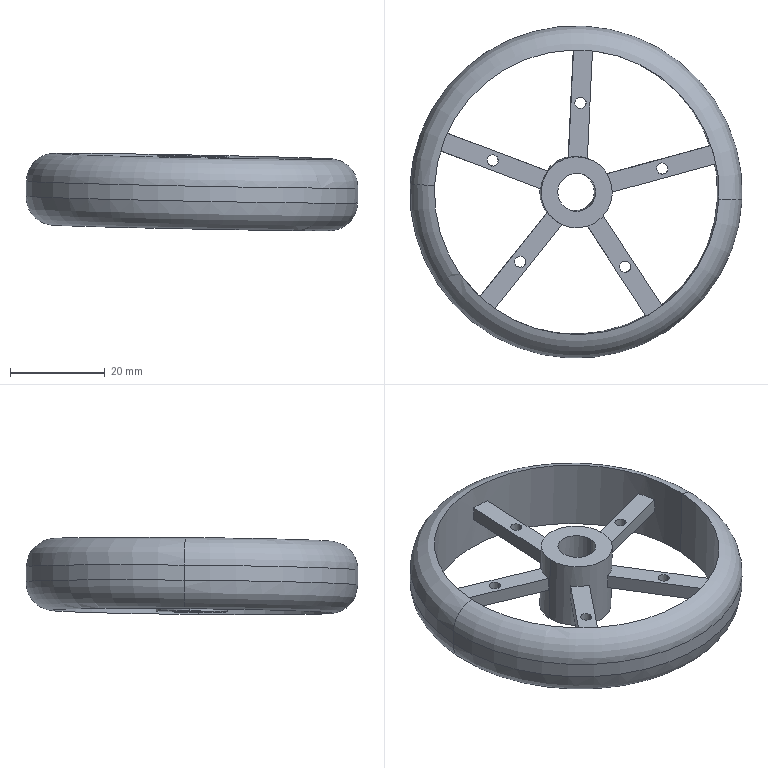Component | SolidWorks | Tire-1 | 1 solid | 44 faces | volume 15414 mm3 | plane 22 | cylinder 18 | torus 4 | commonest cylinder face diameters 2.368 x10 8 x2 70 x2 15 x2 60 x2